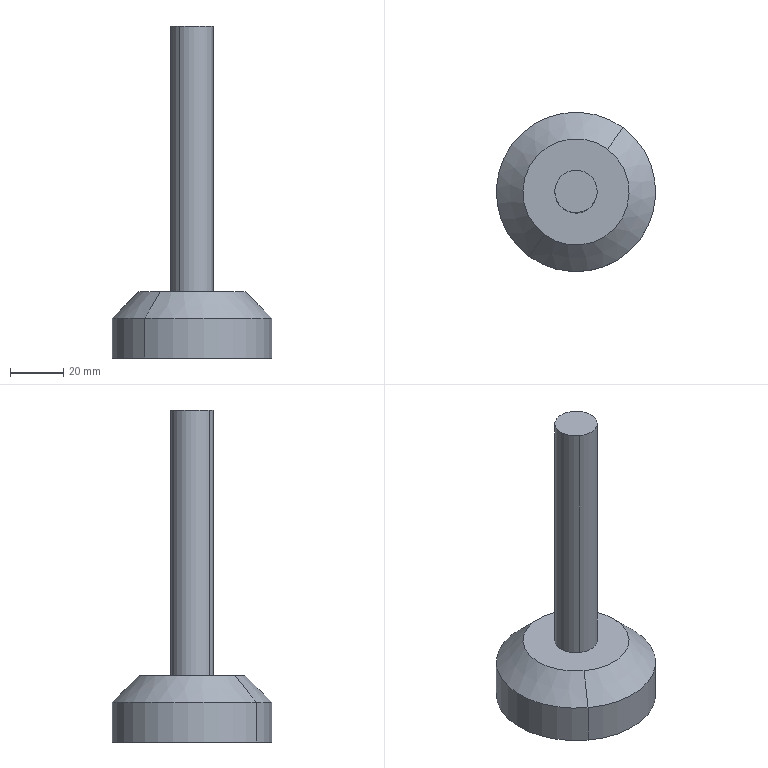Component | SolidWorks | AssemblyVibratoryFeederChassis-1_FootPad-2 | 1 solid | 9 faces | box 60 x 60 x 125 mm | volume 82414 mm3 | cylinder 4 | plane 3 | cone 2 | commonest cylinder face diameters 16 x2 60 x2
build123d program:
from build123d import *

# Parameters (mm, degrees)
SKETCH2_R      = 30
EXTRUDE1_DEPTH = 25
SKETCH3_R      = 8
EXTRUDE2_DEPTH = 100
CHAMFER2_SIZE  = 10


with BuildPart() as part:
    # Sketch2 → Extrude1 (new body)
    with BuildSketch(Plane.XY):
        Circle(SKETCH2_R)
    extrude(amount=-EXTRUDE1_DEPTH)

    # Sketch3 → Extrude2 (add)
    with BuildSketch(Plane.XY):
        Circle(SKETCH3_R)
    extrude(amount=EXTRUDE2_DEPTH)

    # Chamfer2
    chamfer2_edges = [part.edges().sort_by_distance(p)[0] for p in [
        (-30, 0, 0),
    ]]
    chamfer(chamfer2_edges, length=CHAMFER2_SIZE)


solid = part.part

# Placed as in the assembly
solid = solid.moved(Location((-387.449, 248.824, -142), (0, 0, 0)))
STEP:
#1=CARTESIAN_POINT('',(-14.787,10.431,-5.591));
#2=VERTEX_POINT('',#1);
#3=CARTESIAN_POINT('',(-15.72,9.162,-5.591));
#4=VERTEX_POINT('',#3);
#5=CARTESIAN_POINT('',(-15.254,9.796,-5.591));
#6=DIRECTION('',(0.,-0.,1.));
#7=DIRECTION('',(0.5924,0.8056,0.));
#8=AXIS2_PLACEMENT_3D('',#5,#6,#7);
#9=CIRCLE('',#8,0.7874);
#10=EDGE_CURVE('',#2,#4,#9,.T.);
#11=ORIENTED_EDGE('',*,*,#10,.F.);
#12=CARTESIAN_POINT('',(-14.554,10.748,-5.984));
#13=VERTEX_POINT('',#12);
#14=CARTESIAN_POINT('',(-14.787,10.431,-5.591));
#15=DIRECTION('',(0.4189,0.5697,-0.7071));
#16=VECTOR('',#15,39.37);
#17=LINE('',#14,#16);
#18=EDGE_CURVE('',#2,#13,#17,.T.);
#19=ORIENTED_EDGE('',*,*,#18,.T.);
#20=CARTESIAN_POINT('',(-15.954,8.845,-5.984));
#21=VERTEX_POINT('',#20);
#22=CARTESIAN_POINT('',(-15.254,9.796,-5.984));
#23=DIRECTION('',(-0.,0.,-1.));
#24=DIRECTION('',(0.5924,0.8056,0.));
#25=AXIS2_PLACEMENT_3D('',#22,#23,#24);
#26=CIRCLE('',#25,1.181);
#27=EDGE_CURVE('',#21,#13,#26,.T.);
#28=ORIENTED_EDGE('',*,*,#27,.F.);
#29=CARTESIAN_POINT('',(-15.72,9.162,-5.591));
#30=DIRECTION('',(-0.4189,-0.5697,-0.7071));
#31=VECTOR('',#30,39.37);
#32=LINE('',#29,#31);
#33=EDGE_CURVE('',#4,#21,#32,.T.);
#34=ORIENTED_EDGE('',*,*,#33,.F.);
#35=EDGE_LOOP('',(#11,#19,#28,#34));
#36=FACE_OUTER_BOUND('',#35,.T.);
#37=CARTESIAN_POINT('',(-15.254,9.796,-5.591));
#38=DIRECTION('',(-0.,0.,-1.));
#39=DIRECTION('',(-0.5924,-0.8056,0.));
#40=AXIS2_PLACEMENT_3D('',#37,#38,#39);
#41=CONICAL_SURFACE('',#40,0.7874,0.7854);
#42=ADVANCED_FACE('',(#36),#41,.T.);
#43=CARTESIAN_POINT('',(-15.067,10.05,-1.654));
#44=VERTEX_POINT('',#43);
#45=CARTESIAN_POINT('',(-15.44,9.542,-1.654));
#46=VERTEX_POINT('',#45);
#47=CARTESIAN_POINT('',(-15.254,9.796,-1.654));
#48=DIRECTION('',(0.,-0.,1.));
#49=DIRECTION('',(0.5924,0.8056,0.));
#50=AXIS2_PLACEMENT_3D('',#47,#48,#49);
#51=CIRCLE('',#50,0.315);
#52=EDGE_CURVE('',#44,#46,#51,.T.);
#53=ORIENTED_EDGE('',*,*,#52,.F.);
#54=CARTESIAN_POINT('',(-15.067,10.05,-5.591));
#55=VERTEX_POINT('',#54);
#56=CARTESIAN_POINT('',(-15.067,10.05,-1.654));
#57=DIRECTION('',(-0.,0.,-1.));
#58=VECTOR('',#57,39.37);
#59=LINE('',#56,#58);
#60=EDGE_CURVE('',#44,#55,#59,.T.);
#61=ORIENTED_EDGE('',*,*,#60,.T.);
#62=CARTESIAN_POINT('',(-15.44,9.542,-5.591));
#63=VERTEX_POINT('',#62);
#64=CARTESIAN_POINT('',(-15.254,9.796,-5.591));
#65=DIRECTION('',(0.,-0.,1.));
#66=DIRECTION('',(0.5924,0.8056,0.));
#67=AXIS2_PLACEMENT_3D('',#64,#65,#66);
#68=CIRCLE('',#67,0.315);
#69=EDGE_CURVE('',#55,#63,#68,.T.);
#70=ORIENTED_EDGE('',*,*,#69,.T.);
#71=CARTESIAN_POINT('',(-15.44,9.542,-1.654));
#72=DIRECTION('',(-0.,0.,-1.));
#73=VECTOR('',#72,39.37);
#74=LINE('',#71,#73);
#75=EDGE_CURVE('',#46,#63,#74,.T.);
#76=ORIENTED_EDGE('',*,*,#75,.F.);
#77=EDGE_LOOP('',(#53,#61,#70,#76));
#78=FACE_OUTER_BOUND('',#77,.T.);
#79=CARTESIAN_POINT('',(-15.254,9.796,-1.654));
#80=DIRECTION('',(-0.,0.,-1.));
#81=DIRECTION('',(-0.5924,-0.8056,0.));
#82=AXIS2_PLACEMENT_3D('',#79,#80,#81);
#83=CYLINDRICAL_SURFACE('',#82,0.315);
#84=ADVANCED_FACE('',(#78),#83,.T.);
#85=CARTESIAN_POINT('',(-14.554,10.748,-6.575));
#86=VERTEX_POINT('',#85);
#87=CARTESIAN_POINT('',(-15.954,8.845,-6.575));
#88=VERTEX_POINT('',#87);
#89=CARTESIAN_POINT('',(-15.254,9.796,-6.575));
#90=DIRECTION('',(0.,-0.,1.));
#91=DIRECTION('',(0.5924,0.8056,0.));
#92=AXIS2_PLACEMENT_3D('',#89,#90,#91);
#93=CIRCLE('',#92,1.181);
#94=EDGE_CURVE('',#86,#88,#93,.T.);
#95=ORIENTED_EDGE('',*,*,#94,.T.);
#96=CARTESIAN_POINT('',(-15.954,8.845,-6.575));
#97=DIRECTION('',(0.,-0.,1.));
#98=VECTOR('',#97,39.37);
#99=LINE('',#96,#98);
#100=EDGE_CURVE('',#88,#21,#99,.T.);
#101=ORIENTED_EDGE('',*,*,#100,.T.);
#102=ORIENTED_EDGE('',*,*,#27,.T.);
#103=CARTESIAN_POINT('',(-14.554,10.748,-6.575));
#104=DIRECTION('',(0.,-0.,1.));
#105=VECTOR('',#104,39.37);
#106=LINE('',#103,#105);
#107=EDGE_CURVE('',#86,#13,#106,.T.);
#108=ORIENTED_EDGE('',*,*,#107,.F.);
#109=EDGE_LOOP('',(#95,#101,#102,#108));
#110=FACE_OUTER_BOUND('',#109,.T.);
#111=CARTESIAN_POINT('',(-15.254,9.796,-6.575));
#112=DIRECTION('',(0.,-0.,1.));
#113=DIRECTION('',(0.5924,0.8056,0.));
#114=AXIS2_PLACEMENT_3D('',#111,#112,#113);
#115=CYLINDRICAL_SURFACE('',#114,1.181);
#116=ADVANCED_FACE('',(#110),#115,.T.);
#117=CARTESIAN_POINT('',(-15.254,9.796,-5.591));
#118=DIRECTION('',(0.,-0.,1.));
#119=DIRECTION('',(0.5924,0.8056,0.));
#120=AXIS2_PLACEMENT_3D('',#117,#118,#119);
#121=CIRCLE('',#120,0.7874);
#122=EDGE_CURVE('',#4,#2,#121,.T.);
#123=ORIENTED_EDGE('',*,*,#122,.T.);
#124=ORIENTED_EDGE('',*,*,#10,.T.);
#125=EDGE_LOOP('',(#123,#124));
#126=FACE_OUTER_BOUND('',#125,.T.);
#127=CARTESIAN_POINT('',(-15.254,9.796,-5.591));
#128=DIRECTION('',(0.,-0.,1.));
#129=DIRECTION('',(0.5924,0.8056,0.));
#130=AXIS2_PLACEMENT_3D('',#127,#128,#129);
#131=CIRCLE('',#130,0.315);
#132=EDGE_CURVE('',#63,#55,#131,.T.);
#133=ORIENTED_EDGE('',*,*,#132,.F.);
#134=ORIENTED_EDGE('',*,*,#69,.F.);
#135=EDGE_LOOP('',(#133,#134));
#136=FACE_BOUND('',#135,.T.);
#137=CARTESIAN_POINT('',(-15.254,9.796,-5.591));
#138=DIRECTION('',(0.,-0.,1.));
#139=DIRECTION('',(0.5924,0.8056,-0.));
#140=AXIS2_PLACEMENT_3D('',#137,#138,#139);
#141=PLANE('',#140);
#142=ADVANCED_FACE('',(#126,#136),#141,.T.);
#143=ORIENTED_EDGE('',*,*,#100,.F.);
#144=CARTESIAN_POINT('',(-15.254,9.796,-6.575));
#145=DIRECTION('',(0.,-0.,1.));
#146=DIRECTION('',(0.5924,0.8056,0.));
#147=AXIS2_PLACEMENT_3D('',#144,#145,#146);
#148=CIRCLE('',#147,1.181);
#149=EDGE_CURVE('',#88,#86,#148,.T.);
#150=ORIENTED_EDGE('',*,*,#149,.T.);
#151=ORIENTED_EDGE('',*,*,#107,.T.);
#152=CARTESIAN_POINT('',(-15.254,9.796,-5.984));
#153=DIRECTION('',(-0.,0.,-1.));
#154=DIRECTION('',(0.5924,0.8056,0.));
#155=AXIS2_PLACEMENT_3D('',#152,#153,#154);
#156=CIRCLE('',#155,1.181);
#157=EDGE_CURVE('',#13,#21,#156,.T.);
#158=ORIENTED_EDGE('',*,*,#157,.T.);
#159=EDGE_LOOP('',(#143,#150,#151,#158));
#160=FACE_OUTER_BOUND('',#159,.T.);
#161=CARTESIAN_POINT('',(-15.254,9.796,-6.575));
#162=DIRECTION('',(0.,-0.,1.));
#163=DIRECTION('',(0.5924,0.8056,0.));
#164=AXIS2_PLACEMENT_3D('',#161,#162,#163);
#165=CYLINDRICAL_SURFACE('',#164,1.181);
#166=ADVANCED_FACE('',(#160),#165,.T.);
#167=ORIENTED_EDGE('',*,*,#94,.F.);
#168=ORIENTED_EDGE('',*,*,#149,.F.);
#169=EDGE_LOOP('',(#167,#168));
#170=FACE_OUTER_BOUND('',#169,.T.);
#171=CARTESIAN_POINT('',(-15.254,9.796,-6.575));
#172=DIRECTION('',(0.,-0.,1.));
#173=DIRECTION('',(0.5924,0.8056,-0.));
#174=AXIS2_PLACEMENT_3D('',#171,#172,#173);
#175=PLANE('',#174);
#176=ADVANCED_FACE('',(#170),#175,.F.);
#177=ORIENTED_EDGE('',*,*,#60,.F.);
#178=CARTESIAN_POINT('',(-15.254,9.796,-1.654));
#179=DIRECTION('',(0.,-0.,1.));
#180=DIRECTION('',(0.5924,0.8056,0.));
#181=AXIS2_PLACEMENT_3D('',#178,#179,#180);
#182=CIRCLE('',#181,0.315);
#183=EDGE_CURVE('',#46,#44,#182,.T.);
#184=ORIENTED_EDGE('',*,*,#183,.F.);
#185=ORIENTED_EDGE('',*,*,#75,.T.);
#186=ORIENTED_EDGE('',*,*,#132,.T.);
#187=EDGE_LOOP('',(#177,#184,#185,#186));
#188=FACE_OUTER_BOUND('',#187,.T.);
#189=CARTESIAN_POINT('',(-15.254,9.796,-1.654));
#190=DIRECTION('',(-0.,0.,-1.));
#191=DIRECTION('',(-0.5924,-0.8056,0.));
#192=AXIS2_PLACEMENT_3D('',#189,#190,#191);
#193=CYLINDRICAL_SURFACE('',#192,0.315);
#194=ADVANCED_FACE('',(#188),#193,.T.);
#195=ORIENTED_EDGE('',*,*,#183,.T.);
#196=ORIENTED_EDGE('',*,*,#52,.T.);
#197=EDGE_LOOP('',(#195,#196));
#198=FACE_OUTER_BOUND('',#197,.T.);
#199=CARTESIAN_POINT('',(-15.254,9.796,-1.654));
#200=DIRECTION('',(0.,-0.,1.));
#201=DIRECTION('',(0.5924,0.8056,-0.));
#202=AXIS2_PLACEMENT_3D('',#199,#200,#201);
#203=PLANE('',#202);
#204=ADVANCED_FACE('',(#198),#203,.T.);
#205=ORIENTED_EDGE('',*,*,#18,.F.);
#206=ORIENTED_EDGE('',*,*,#122,.F.);
#207=ORIENTED_EDGE('',*,*,#33,.T.);
#208=ORIENTED_EDGE('',*,*,#157,.F.);
#209=EDGE_LOOP('',(#205,#206,#207,#208));
#210=FACE_OUTER_BOUND('',#209,.T.);
#211=CARTESIAN_POINT('',(-15.254,9.796,-5.591));
#212=DIRECTION('',(-0.,0.,-1.));
#213=DIRECTION('',(-0.5924,-0.8056,0.));
#214=AXIS2_PLACEMENT_3D('',#211,#212,#213);
#215=CONICAL_SURFACE('',#214,0.7874,0.7854);
#216=ADVANCED_FACE('',(#210),#215,.T.);
#217=CLOSED_SHELL('',(#42,#84,#116,#142,#166,#176,#194,#204,#216));
#218=MANIFOLD_SOLID_BREP('',#217);
#219=CARTESIAN_POINT('',(0.,0.,0.));
#220=DIRECTION('',(0.,0.,1.));
#221=DIRECTION('',(1.,0.,0.));
#222=AXIS2_PLACEMENT_3D('',#219,#220,#221);
#223=(LENGTH_UNIT()NAMED_UNIT(*)SI_UNIT($,.METRE.));
#224=LENGTH_MEASURE_WITH_UNIT(LENGTH_MEASURE(0.0254),#223);
#225=DIMENSIONAL_EXPONENTS(1.,0.,0.,0.,0.,0.,0.);
#226=(CONVERSION_BASED_UNIT('',#224)LENGTH_UNIT()NAMED_UNIT(#225));
#227=UNCERTAINTY_MEASURE_WITH_UNIT(LENGTH_MEASURE(0.00001),#226,'','');
#228=(NAMED_UNIT(*)PLANE_ANGLE_UNIT()SI_UNIT($,.RADIAN.));
#229=(NAMED_UNIT(*)SI_UNIT($,.STERADIAN.)SOLID_ANGLE_UNIT());
#230=(GEOMETRIC_REPRESENTATION_CONTEXT(3)GLOBAL_UNCERTAINTY_ASSIGNED_CONTEXT((#227))GLOBAL_UNIT_ASSIGNED_CONTEXT((#226,#228,#229))REPRESENTATION_CONTEXT('',''));
#231=ADVANCED_BREP_SHAPE_REPRESENTATION('',(#218,#222),#230);
#232=COLOUR_RGB('',0.7922,0.8196,0.9333);
#233=FILL_AREA_STYLE_COLOUR('',#232);
#234=FILL_AREA_STYLE('',(#233));
#235=SURFACE_STYLE_FILL_AREA(#234);
#236=SURFACE_SIDE_STYLE('',(#235));
#237=SURFACE_STYLE_USAGE(.BOTH.,#236);
#238=PRESENTATION_STYLE_ASSIGNMENT((#237));
#239=STYLED_ITEM('',(#238),#218);
#240=PRESENTATION_LAYER_ASSIGNMENT('','',(#239));
#241=(LENGTH_UNIT()NAMED_UNIT(*)SI_UNIT($,.METRE.));
#242=LENGTH_MEASURE_WITH_UNIT(LENGTH_MEASURE(0.0254),#241);
#243=DIMENSIONAL_EXPONENTS(1.,0.,0.,0.,0.,0.,0.);
#244=(CONVERSION_BASED_UNIT('',#242)LENGTH_UNIT()NAMED_UNIT(#243));
#245=UNCERTAINTY_MEASURE_WITH_UNIT(LENGTH_MEASURE(0.00001),#244,'','');
#246=(NAMED_UNIT(*)PLANE_ANGLE_UNIT()SI_UNIT($,.RADIAN.));
#247=(NAMED_UNIT(*)SI_UNIT($,.STERADIAN.)SOLID_ANGLE_UNIT());
#248=(GEOMETRIC_REPRESENTATION_CONTEXT(3)GLOBAL_UNCERTAINTY_ASSIGNED_CONTEXT((#245))GLOBAL_UNIT_ASSIGNED_CONTEXT((#244,#246,#247))REPRESENTATION_CONTEXT('',''));
#249=MECHANICAL_DESIGN_GEOMETRIC_PRESENTATION_REPRESENTATION('',(#239),#248);